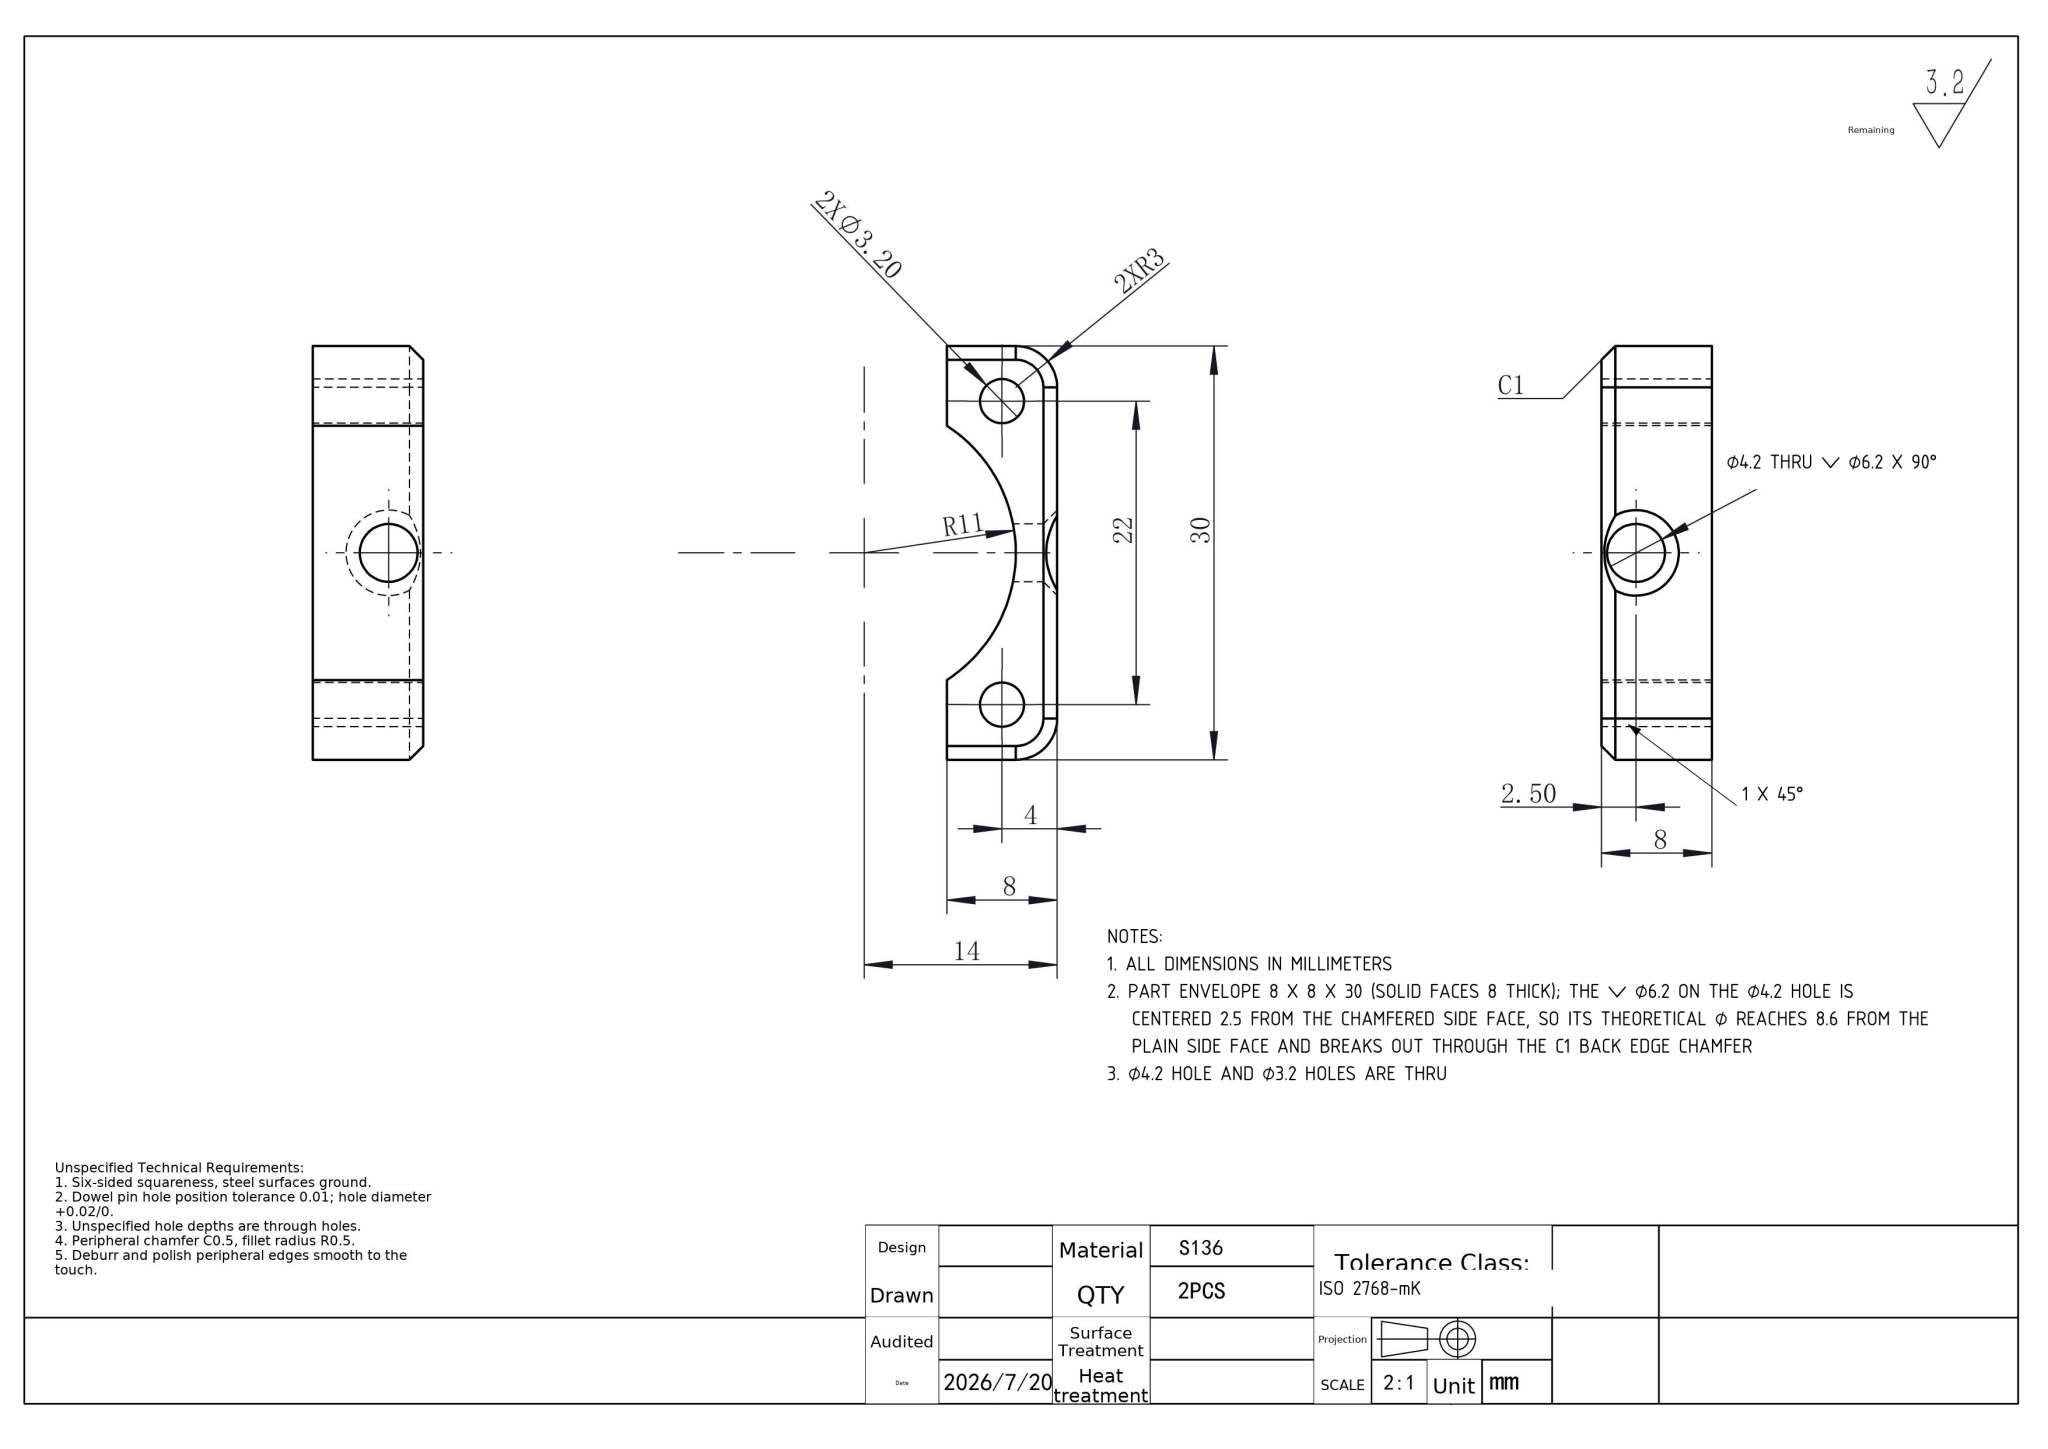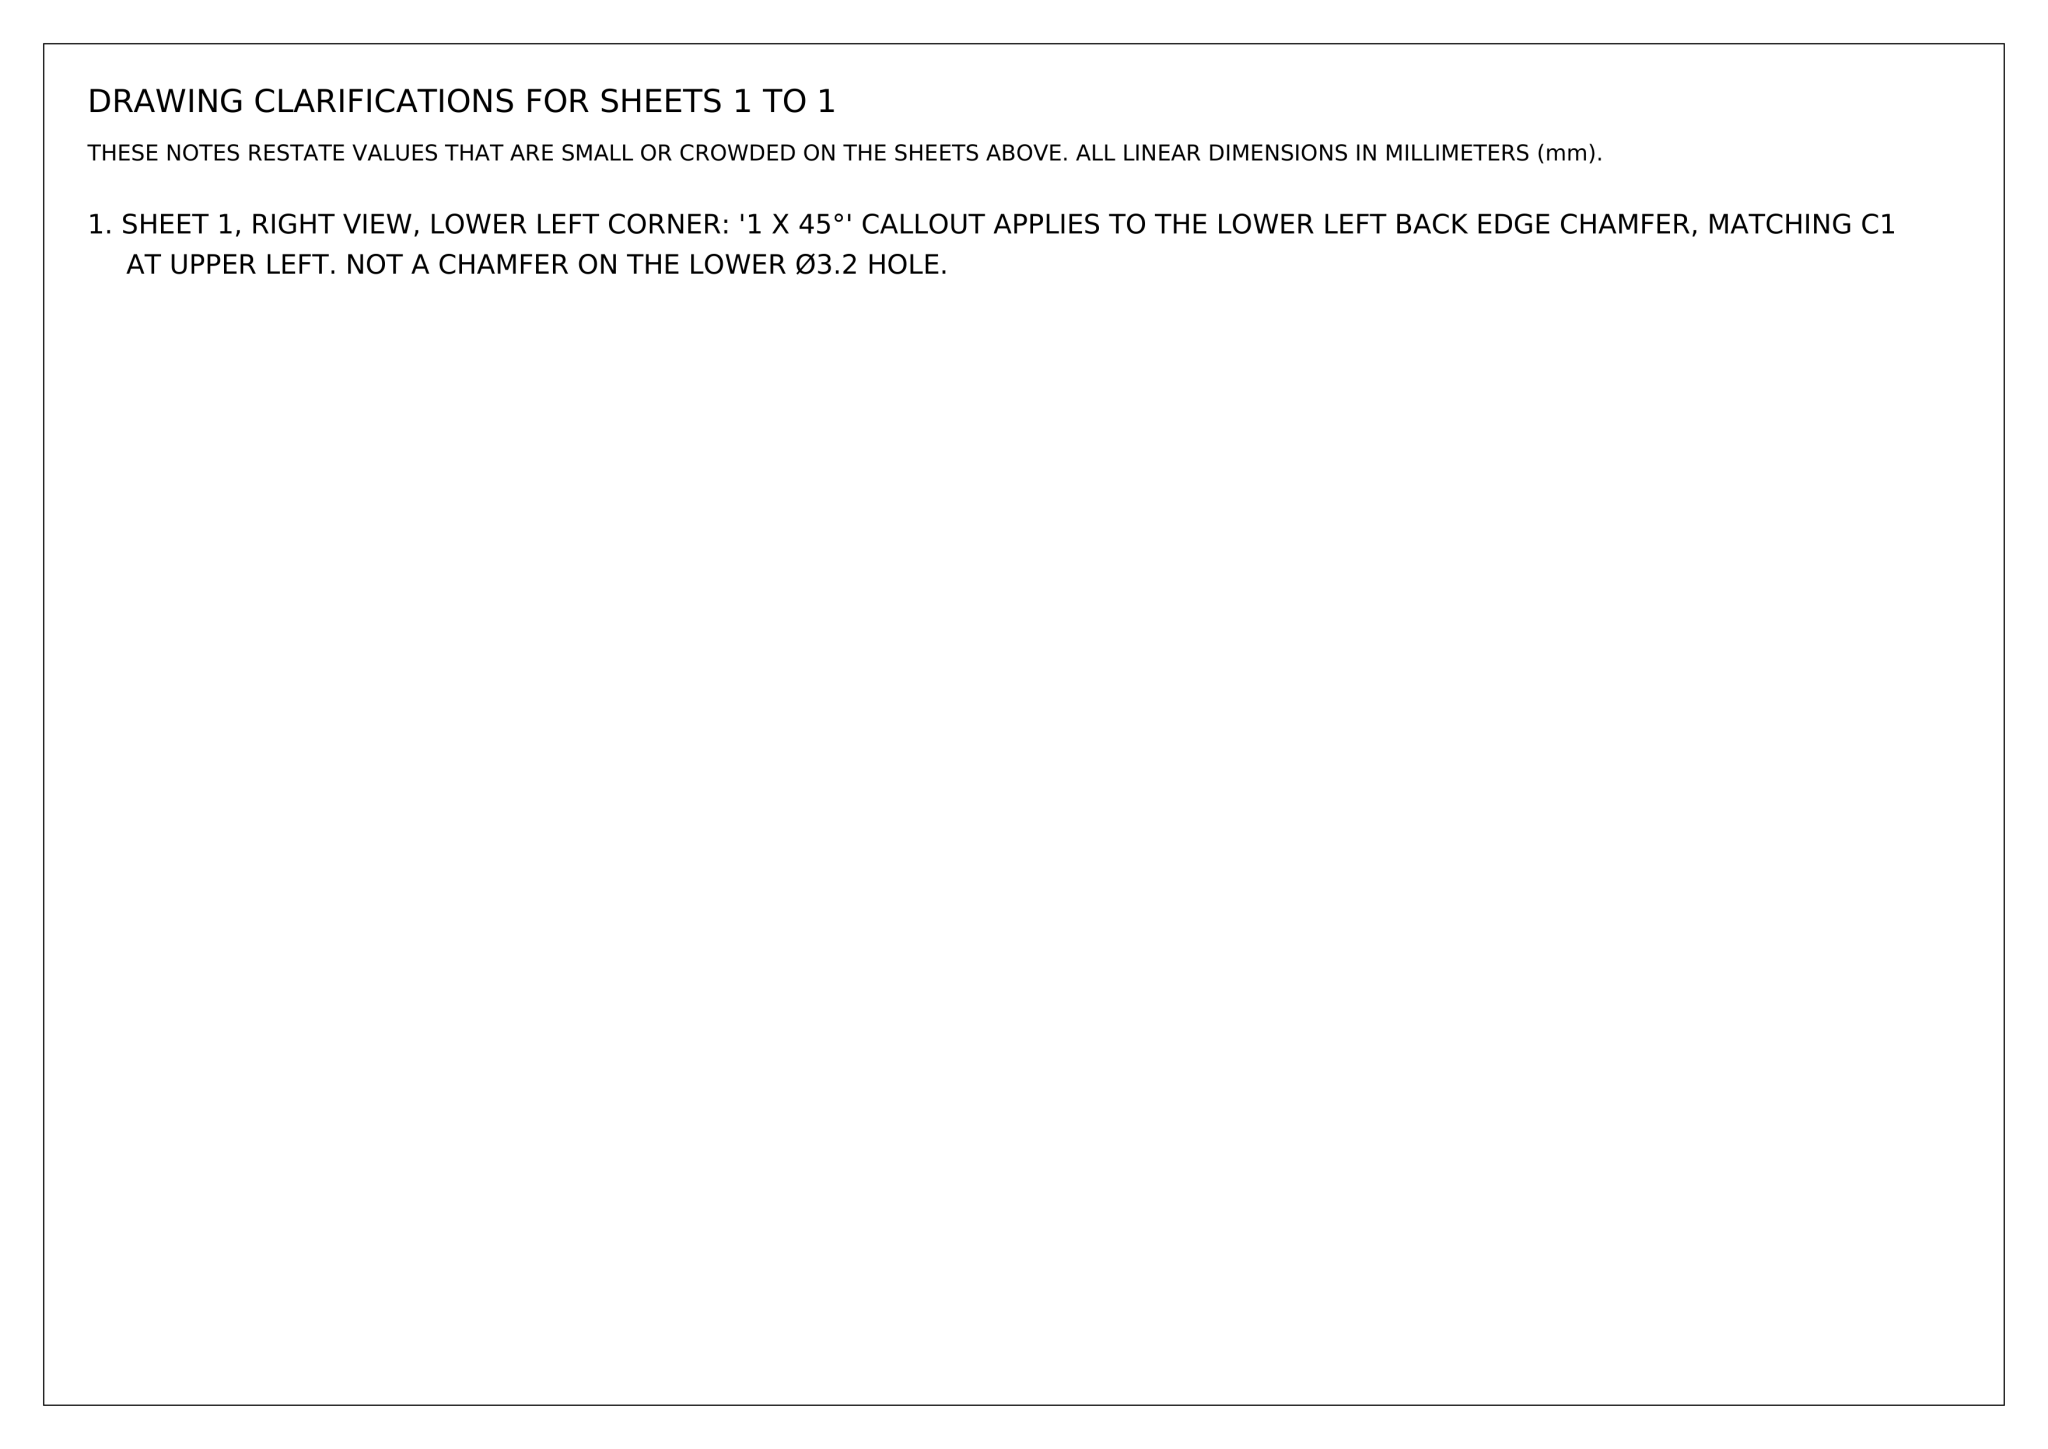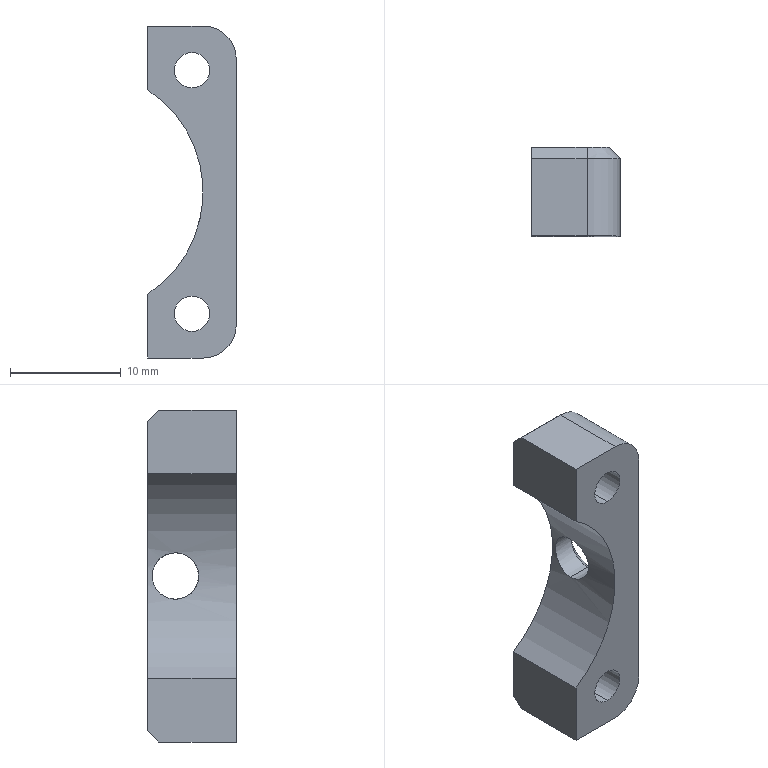Part | NX | mm | 1 solid | 23 faces | box 8 x 8 x 30 mm | volume 1172 mm3 | plane 10 | cylinder 9 | cone 4 | commonest cylinder face diameters 3.2 x4 4.2 x2 6 x2 22 x1
STEP:
#1=COLOUR_RGB('',0.7922,0.8196,0.9333);
#2=FILL_AREA_STYLE_COLOUR('',#1);
#3=FILL_AREA_STYLE('',(#2));
#4=SURFACE_STYLE_FILL_AREA(#3);
#5=SURFACE_SIDE_STYLE('',(#4));
#6=SURFACE_STYLE_USAGE(.BOTH.,#5);
#7=PRESENTATION_STYLE_ASSIGNMENT((#6));
#8=CARTESIAN_POINT('',(13.,5.5,2.1));
#9=VERTEX_POINT('',#8);
#10=CARTESIAN_POINT('',(13.,5.5,-2.1));
#11=VERTEX_POINT('',#10);
#12=CARTESIAN_POINT('',(13.,5.5,0.));
#13=DIRECTION('',(1.,0.,0.));
#14=DIRECTION('',(0.,0.,1.));
#15=AXIS2_PLACEMENT_3D('',#12,#13,#14);
#16=CIRCLE('',#15,2.1);
#17=EDGE_CURVE('',#9,#11,#16,.T.);
#18=ORIENTED_EDGE('',*,*,#17,.F.);
#19=CARTESIAN_POINT('',(14.,5.5,3.1));
#20=VERTEX_POINT('',#19);
#21=CARTESIAN_POINT('',(13.,5.5,2.1));
#22=DIRECTION('',(0.7071,0.,0.7071));
#23=VECTOR('',#22,1000.);
#24=LINE('',#21,#23);
#25=EDGE_CURVE('',#9,#20,#24,.T.);
#26=ORIENTED_EDGE('',*,*,#25,.T.);
#27=CARTESIAN_POINT('',(14.,5.5,-3.1));
#28=VERTEX_POINT('',#27);
#29=CARTESIAN_POINT('',(14.,5.5,0.));
#30=DIRECTION('',(-1.,0.,0.));
#31=DIRECTION('',(0.,0.,1.));
#32=AXIS2_PLACEMENT_3D('',#29,#30,#31);
#33=CIRCLE('',#32,3.1);
#34=EDGE_CURVE('',#28,#20,#33,.T.);
#35=ORIENTED_EDGE('',*,*,#34,.F.);
#36=CARTESIAN_POINT('',(13.,5.5,-2.1));
#37=DIRECTION('',(0.7071,0.,-0.7071));
#38=VECTOR('',#37,1000.);
#39=LINE('',#36,#38);
#40=EDGE_CURVE('',#11,#28,#39,.T.);
#41=ORIENTED_EDGE('',*,*,#40,.F.);
#42=EDGE_LOOP('',(#18,#26,#35,#41));
#43=FACE_OUTER_BOUND('',#42,.T.);
#44=CARTESIAN_POINT('',(13.,5.5,0.));
#45=DIRECTION('',(1.,0.,0.));
#46=DIRECTION('',(0.,0.,-1.));
#47=AXIS2_PLACEMENT_3D('',#44,#45,#46);
#48=CONICAL_SURFACE('',#47,2.1,0.7854);
#49=ADVANCED_FACE('',(#43),#48,.F.);
#50=CARTESIAN_POINT('',(10.798,5.5,2.1));
#51=VERTEX_POINT('',#50);
#52=CARTESIAN_POINT('',(10.798,5.5,-2.1));
#53=VERTEX_POINT('',#52);
#54=CARTESIAN_POINT('',(10.798,5.5,2.1));
#55=CARTESIAN_POINT('',(10.798,5.226,2.1));
#56=CARTESIAN_POINT('',(10.809,4.949,2.045));
#57=CARTESIAN_POINT('',(10.837,4.57,1.888));
#58=CARTESIAN_POINT('',(10.848,4.447,1.822));
#59=CARTESIAN_POINT('',(10.873,4.218,1.669));
#60=CARTESIAN_POINT('',(10.886,4.113,1.583));
#61=CARTESIAN_POINT('',(10.912,3.919,1.389));
#62=CARTESIAN_POINT('',(10.926,3.831,1.281));
#63=CARTESIAN_POINT('',(10.95,3.678,1.054));
#64=CARTESIAN_POINT('',(10.961,3.614,0.9335));
#65=CARTESIAN_POINT('',(10.989,3.455,0.5515));
#66=CARTESIAN_POINT('',(11.,3.4,0.2784));
#67=CARTESIAN_POINT('',(11.,3.4,-0.1376));
#68=CARTESIAN_POINT('',(10.997,3.413,-0.2741));
#69=CARTESIAN_POINT('',(10.987,3.467,-0.5432));
#70=CARTESIAN_POINT('',(10.98,3.507,-0.677));
#71=CARTESIAN_POINT('',(10.961,3.613,-0.9308));
#72=CARTESIAN_POINT('',(10.95,3.677,-1.051));
#73=CARTESIAN_POINT('',(10.926,3.829,-1.28));
#74=CARTESIAN_POINT('',(10.913,3.918,-1.387));
#75=CARTESIAN_POINT('',(10.873,4.207,-1.677));
#76=CARTESIAN_POINT('',(10.847,4.441,-1.834));
#77=CARTESIAN_POINT('',(10.818,4.819,-1.991));
#78=CARTESIAN_POINT('',(10.811,4.953,-2.032));
#79=CARTESIAN_POINT('',(10.8,5.224,-2.086));
#80=CARTESIAN_POINT('',(10.798,5.361,-2.1));
#81=CARTESIAN_POINT('',(10.798,5.5,-2.1));
#82=B_SPLINE_CURVE_WITH_KNOTS('',3,(#54,#55,#56,#57,#58,#59,#60,#61,#62,#63,#64,#65,#66,#67,#68,#69,#70,#71,#72,#73,#74,#75,#76,#77,#78,#79,#80,#81),.UNSPECIFIED.,.F.,.F.,(4,2,2,2,2,2,2,2,2,2,2,2,2,4),(0.006581,0.007403,0.007814,0.008225,0.008637,0.009048,0.00987,0.01028,0.01069,0.0111,0.01151,0.01234,0.01275,0.01316),.UNSPECIFIED.);
#83=EDGE_CURVE('',#51,#53,#82,.T.);
#84=ORIENTED_EDGE('',*,*,#83,.F.);
#85=CARTESIAN_POINT('',(6.,5.5,2.1));
#86=DIRECTION('',(1.,0.,0.));
#87=VECTOR('',#86,1000.);
#88=LINE('',#85,#87);
#89=EDGE_CURVE('',#51,#9,#88,.T.);
#90=ORIENTED_EDGE('',*,*,#89,.T.);
#91=ORIENTED_EDGE('',*,*,#17,.T.);
#92=CARTESIAN_POINT('',(6.,5.5,-2.1));
#93=DIRECTION('',(1.,0.,0.));
#94=VECTOR('',#93,1000.);
#95=LINE('',#92,#94);
#96=EDGE_CURVE('',#53,#11,#95,.T.);
#97=ORIENTED_EDGE('',*,*,#96,.F.);
#98=EDGE_LOOP('',(#84,#90,#91,#97));
#99=FACE_OUTER_BOUND('',#98,.T.);
#100=CARTESIAN_POINT('',(6.,5.5,0.));
#101=DIRECTION('',(1.,0.,0.));
#102=DIRECTION('',(0.,0.,-1.));
#103=AXIS2_PLACEMENT_3D('',#100,#101,#102);
#104=CYLINDRICAL_SURFACE('',#103,2.1);
#105=ADVANCED_FACE('',(#99),#104,.F.);
#106=CARTESIAN_POINT('',(10.,0.,-12.6));
#107=VERTEX_POINT('',#106);
#108=CARTESIAN_POINT('',(10.,0.,-9.4));
#109=VERTEX_POINT('',#108);
#110=CARTESIAN_POINT('',(10.,0.,-11.));
#111=DIRECTION('',(0.,1.,0.));
#112=DIRECTION('',(0.,0.,1.));
#113=AXIS2_PLACEMENT_3D('',#110,#111,#112);
#114=CIRCLE('',#113,1.6);
#115=EDGE_CURVE('',#107,#109,#114,.T.);
#116=ORIENTED_EDGE('',*,*,#115,.F.);
#117=CARTESIAN_POINT('',(10.,8.,-12.6));
#118=VERTEX_POINT('',#117);
#119=CARTESIAN_POINT('',(10.,0.,-12.6));
#120=DIRECTION('',(0.,1.,0.));
#121=VECTOR('',#120,1000.);
#122=LINE('',#119,#121);
#123=EDGE_CURVE('',#107,#118,#122,.T.);
#124=ORIENTED_EDGE('',*,*,#123,.T.);
#125=CARTESIAN_POINT('',(10.,8.,-9.4));
#126=VERTEX_POINT('',#125);
#127=CARTESIAN_POINT('',(10.,8.,-11.));
#128=DIRECTION('',(0.,1.,0.));
#129=DIRECTION('',(0.,0.,1.));
#130=AXIS2_PLACEMENT_3D('',#127,#128,#129);
#131=CIRCLE('',#130,1.6);
#132=EDGE_CURVE('',#118,#126,#131,.T.);
#133=ORIENTED_EDGE('',*,*,#132,.T.);
#134=CARTESIAN_POINT('',(10.,0.,-9.4));
#135=DIRECTION('',(0.,1.,0.));
#136=VECTOR('',#135,1000.);
#137=LINE('',#134,#136);
#138=EDGE_CURVE('',#109,#126,#137,.T.);
#139=ORIENTED_EDGE('',*,*,#138,.F.);
#140=EDGE_LOOP('',(#116,#124,#133,#139));
#141=FACE_OUTER_BOUND('',#140,.T.);
#142=CARTESIAN_POINT('',(10.,0.,-11.));
#143=DIRECTION('',(0.,1.,0.));
#144=DIRECTION('',(0.,0.,1.));
#145=AXIS2_PLACEMENT_3D('',#142,#143,#144);
#146=CYLINDRICAL_SURFACE('',#145,1.6);
#147=ADVANCED_FACE('',(#141),#146,.F.);
#148=CARTESIAN_POINT('',(10.,0.,9.4));
#149=VERTEX_POINT('',#148);
#150=CARTESIAN_POINT('',(10.,0.,12.6));
#151=VERTEX_POINT('',#150);
#152=CARTESIAN_POINT('',(10.,0.,11.));
#153=DIRECTION('',(0.,1.,0.));
#154=DIRECTION('',(0.,0.,1.));
#155=AXIS2_PLACEMENT_3D('',#152,#153,#154);
#156=CIRCLE('',#155,1.6);
#157=EDGE_CURVE('',#149,#151,#156,.T.);
#158=ORIENTED_EDGE('',*,*,#157,.F.);
#159=CARTESIAN_POINT('',(10.,8.,9.4));
#160=VERTEX_POINT('',#159);
#161=CARTESIAN_POINT('',(10.,0.,9.4));
#162=DIRECTION('',(0.,1.,0.));
#163=VECTOR('',#162,1000.);
#164=LINE('',#161,#163);
#165=EDGE_CURVE('',#149,#160,#164,.T.);
#166=ORIENTED_EDGE('',*,*,#165,.T.);
#167=CARTESIAN_POINT('',(10.,8.,12.6));
#168=VERTEX_POINT('',#167);
#169=CARTESIAN_POINT('',(10.,8.,11.));
#170=DIRECTION('',(0.,1.,0.));
#171=DIRECTION('',(0.,0.,1.));
#172=AXIS2_PLACEMENT_3D('',#169,#170,#171);
#173=CIRCLE('',#172,1.6);
#174=EDGE_CURVE('',#160,#168,#173,.T.);
#175=ORIENTED_EDGE('',*,*,#174,.T.);
#176=CARTESIAN_POINT('',(10.,0.,12.6));
#177=DIRECTION('',(0.,1.,0.));
#178=VECTOR('',#177,1000.);
#179=LINE('',#176,#178);
#180=EDGE_CURVE('',#151,#168,#179,.T.);
#181=ORIENTED_EDGE('',*,*,#180,.F.);
#182=EDGE_LOOP('',(#158,#166,#175,#181));
#183=FACE_OUTER_BOUND('',#182,.T.);
#184=CARTESIAN_POINT('',(10.,0.,11.));
#185=DIRECTION('',(0.,1.,0.));
#186=DIRECTION('',(0.,0.,1.));
#187=AXIS2_PLACEMENT_3D('',#184,#185,#186);
#188=CYLINDRICAL_SURFACE('',#187,1.6);
#189=ADVANCED_FACE('',(#183),#188,.F.);
#190=CARTESIAN_POINT('',(14.,7.,-12.));
#191=VERTEX_POINT('',#190);
#192=CARTESIAN_POINT('',(14.,7.,-2.713));
#193=VERTEX_POINT('',#192);
#194=CARTESIAN_POINT('',(14.,7.,12.));
#195=DIRECTION('',(0.,0.,1.));
#196=VECTOR('',#195,1000.);
#197=LINE('',#194,#196);
#198=EDGE_CURVE('',#191,#193,#197,.T.);
#199=ORIENTED_EDGE('',*,*,#198,.T.);
#200=CARTESIAN_POINT('',(14.,5.5,0.));
#201=DIRECTION('',(-1.,0.,0.));
#202=DIRECTION('',(0.,0.,1.));
#203=AXIS2_PLACEMENT_3D('',#200,#201,#202);
#204=CIRCLE('',#203,3.1);
#205=EDGE_CURVE('',#193,#28,#204,.T.);
#206=ORIENTED_EDGE('',*,*,#205,.T.);
#207=ORIENTED_EDGE('',*,*,#34,.T.);
#208=CARTESIAN_POINT('',(14.,7.,2.713));
#209=VERTEX_POINT('',#208);
#210=CARTESIAN_POINT('',(14.,5.5,0.));
#211=DIRECTION('',(-1.,0.,0.));
#212=DIRECTION('',(0.,0.,1.));
#213=AXIS2_PLACEMENT_3D('',#210,#211,#212);
#214=CIRCLE('',#213,3.1);
#215=EDGE_CURVE('',#20,#209,#214,.T.);
#216=ORIENTED_EDGE('',*,*,#215,.T.);
#217=CARTESIAN_POINT('',(14.,7.,12.));
#218=VERTEX_POINT('',#217);
#219=CARTESIAN_POINT('',(14.,7.,12.));
#220=DIRECTION('',(0.,0.,1.));
#221=VECTOR('',#220,1000.);
#222=LINE('',#219,#221);
#223=EDGE_CURVE('',#209,#218,#222,.T.);
#224=ORIENTED_EDGE('',*,*,#223,.T.);
#225=CARTESIAN_POINT('',(14.,0.,12.));
#226=VERTEX_POINT('',#225);
#227=CARTESIAN_POINT('',(14.,8.,12.));
#228=DIRECTION('',(0.,-1.,0.));
#229=VECTOR('',#228,1000.);
#230=LINE('',#227,#229);
#231=EDGE_CURVE('',#218,#226,#230,.T.);
#232=ORIENTED_EDGE('',*,*,#231,.T.);
#233=CARTESIAN_POINT('',(14.,0.,-12.));
#234=VERTEX_POINT('',#233);
#235=CARTESIAN_POINT('',(14.,0.,-15.));
#236=DIRECTION('',(0.,0.,-1.));
#237=VECTOR('',#236,1000.);
#238=LINE('',#235,#237);
#239=EDGE_CURVE('',#226,#234,#238,.T.);
#240=ORIENTED_EDGE('',*,*,#239,.T.);
#241=CARTESIAN_POINT('',(14.,8.,-12.));
#242=DIRECTION('',(0.,1.,0.));
#243=VECTOR('',#242,1000.);
#244=LINE('',#241,#243);
#245=EDGE_CURVE('',#234,#191,#244,.T.);
#246=ORIENTED_EDGE('',*,*,#245,.T.);
#247=EDGE_LOOP('',(#199,#206,#207,#216,#224,#232,#240,#246));
#248=FACE_OUTER_BOUND('',#247,.T.);
#249=CARTESIAN_POINT('',(14.,8.,-15.));
#250=DIRECTION('',(-1.,0.,0.));
#251=DIRECTION('',(0.,0.,1.));
#252=AXIS2_PLACEMENT_3D('',#249,#250,#251);
#253=PLANE('',#252);
#254=ADVANCED_FACE('',(#248),#253,.F.);
#255=CARTESIAN_POINT('',(6.,7.,-15.));
#256=VERTEX_POINT('',#255);
#257=CARTESIAN_POINT('',(6.,0.,-15.));
#258=VERTEX_POINT('',#257);
#259=CARTESIAN_POINT('',(6.,8.,-15.));
#260=DIRECTION('',(0.,-1.,0.));
#261=VECTOR('',#260,1000.);
#262=LINE('',#259,#261);
#263=EDGE_CURVE('',#256,#258,#262,.T.);
#264=ORIENTED_EDGE('',*,*,#263,.F.);
#265=CARTESIAN_POINT('',(11.,7.,-15.));
#266=VERTEX_POINT('',#265);
#267=CARTESIAN_POINT('',(11.,7.,-15.));
#268=DIRECTION('',(1.,0.,0.));
#269=VECTOR('',#268,1000.);
#270=LINE('',#267,#269);
#271=EDGE_CURVE('',#256,#266,#270,.T.);
#272=ORIENTED_EDGE('',*,*,#271,.T.);
#273=CARTESIAN_POINT('',(11.,0.,-15.));
#274=VERTEX_POINT('',#273);
#275=CARTESIAN_POINT('',(11.,8.,-15.));
#276=DIRECTION('',(0.,-1.,0.));
#277=VECTOR('',#276,1000.);
#278=LINE('',#275,#277);
#279=EDGE_CURVE('',#266,#274,#278,.T.);
#280=ORIENTED_EDGE('',*,*,#279,.T.);
#281=CARTESIAN_POINT('',(6.,0.,-15.));
#282=DIRECTION('',(-1.,0.,0.));
#283=VECTOR('',#282,1000.);
#284=LINE('',#281,#283);
#285=EDGE_CURVE('',#274,#258,#284,.T.);
#286=ORIENTED_EDGE('',*,*,#285,.T.);
#287=EDGE_LOOP('',(#264,#272,#280,#286));
#288=FACE_OUTER_BOUND('',#287,.T.);
#289=CARTESIAN_POINT('',(6.,8.,-15.));
#290=DIRECTION('',(0.,0.,1.));
#291=DIRECTION('',(1.,0.,0.));
#292=AXIS2_PLACEMENT_3D('',#289,#290,#291);
#293=PLANE('',#292);
#294=ADVANCED_FACE('',(#288),#293,.F.);
#295=CARTESIAN_POINT('',(6.,8.,-14.));
#296=VERTEX_POINT('',#295);
#297=CARTESIAN_POINT('',(6.,8.,-9.22));
#298=VERTEX_POINT('',#297);
#299=CARTESIAN_POINT('',(6.,8.,-15.));
#300=DIRECTION('',(0.,0.,1.));
#301=VECTOR('',#300,1000.);
#302=LINE('',#299,#301);
#303=EDGE_CURVE('',#296,#298,#302,.T.);
#304=ORIENTED_EDGE('',*,*,#303,.F.);
#305=CARTESIAN_POINT('',(6.,8.,-14.));
#306=DIRECTION('',(0.,-0.7071,-0.7071));
#307=VECTOR('',#306,1000.);
#308=LINE('',#305,#307);
#309=EDGE_CURVE('',#296,#256,#308,.T.);
#310=ORIENTED_EDGE('',*,*,#309,.T.);
#311=ORIENTED_EDGE('',*,*,#263,.T.);
#312=CARTESIAN_POINT('',(6.,0.,-9.22));
#313=VERTEX_POINT('',#312);
#314=CARTESIAN_POINT('',(6.,0.,-15.));
#315=DIRECTION('',(0.,0.,1.));
#316=VECTOR('',#315,1000.);
#317=LINE('',#314,#316);
#318=EDGE_CURVE('',#258,#313,#317,.T.);
#319=ORIENTED_EDGE('',*,*,#318,.T.);
#320=CARTESIAN_POINT('',(6.,8.,-9.22));
#321=DIRECTION('',(0.,-1.,0.));
#322=VECTOR('',#321,1000.);
#323=LINE('',#320,#322);
#324=EDGE_CURVE('',#298,#313,#323,.T.);
#325=ORIENTED_EDGE('',*,*,#324,.F.);
#326=EDGE_LOOP('',(#304,#310,#311,#319,#325));
#327=FACE_OUTER_BOUND('',#326,.T.);
#328=CARTESIAN_POINT('',(6.,8.,-15.));
#329=DIRECTION('',(1.,0.,0.));
#330=DIRECTION('',(0.,0.,-1.));
#331=AXIS2_PLACEMENT_3D('',#328,#329,#330);
#332=PLANE('',#331);
#333=ADVANCED_FACE('',(#327),#332,.F.);
#334=CARTESIAN_POINT('',(10.798,5.5,-2.1));
#335=CARTESIAN_POINT('',(10.798,5.639,-2.1));
#336=CARTESIAN_POINT('',(10.8,5.776,-2.086));
#337=CARTESIAN_POINT('',(10.811,6.045,-2.033));
#338=CARTESIAN_POINT('',(10.818,6.178,-1.992));
#339=CARTESIAN_POINT('',(10.837,6.432,-1.887));
#340=CARTESIAN_POINT('',(10.848,6.553,-1.822));
#341=CARTESIAN_POINT('',(10.873,6.781,-1.67));
#342=CARTESIAN_POINT('',(10.886,6.889,-1.581));
#343=CARTESIAN_POINT('',(10.926,7.178,-1.291));
#344=CARTESIAN_POINT('',(10.952,7.335,-1.057));
#345=CARTESIAN_POINT('',(10.989,7.544,-0.5523));
#346=CARTESIAN_POINT('',(11.,7.6,-0.2755));
#347=CARTESIAN_POINT('',(11.,7.6,0.1365));
#348=CARTESIAN_POINT('',(10.997,7.586,0.276));
#349=CARTESIAN_POINT('',(10.987,7.533,0.5456));
#350=CARTESIAN_POINT('',(10.98,7.493,0.6767));
#351=CARTESIAN_POINT('',(10.961,7.387,0.9314));
#352=CARTESIAN_POINT('',(10.95,7.322,1.054));
#353=CARTESIAN_POINT('',(10.926,7.17,1.281));
#354=CARTESIAN_POINT('',(10.913,7.082,1.387));
#355=CARTESIAN_POINT('',(10.886,6.887,1.583));
#356=CARTESIAN_POINT('',(10.873,6.781,1.669));
#357=CARTESIAN_POINT('',(10.848,6.554,1.821));
#358=CARTESIAN_POINT('',(10.837,6.431,1.887));
#359=CARTESIAN_POINT('',(10.818,6.177,1.992));
#360=CARTESIAN_POINT('',(10.811,6.046,2.032));
#361=CARTESIAN_POINT('',(10.8,5.777,2.086));
#362=CARTESIAN_POINT('',(10.798,5.637,2.1));
#363=CARTESIAN_POINT('',(10.798,5.5,2.1));
#364=B_SPLINE_CURVE_WITH_KNOTS('',3,(#334,#335,#336,#337,#338,#339,#340,#341,#342,#343,#344,#345,#346,#347,#348,#349,#350,#351,#352,#353,#354,#355,#356,#357,#358,#359,#360,#361,#362,#363),.UNSPECIFIED.,.F.,.F.,(4,2,2,2,2,2,2,2,2,2,2,2,2,2,4),(0.,0.0004113,0.0008226,0.001234,0.001645,0.002468,0.00329,0.003702,0.004113,0.004524,0.004935,0.005347,0.005758,0.006169,0.006581),.UNSPECIFIED.);
#365=EDGE_CURVE('',#53,#51,#364,.T.);
#366=ORIENTED_EDGE('',*,*,#365,.T.);
#367=ORIENTED_EDGE('',*,*,#83,.T.);
#368=EDGE_LOOP('',(#366,#367));
#369=FACE_BOUND('',#368,.T.);
#370=CARTESIAN_POINT('',(6.,0.,9.22));
#371=VERTEX_POINT('',#370);
#372=CARTESIAN_POINT('',(0.,0.,0.));
#373=DIRECTION('',(0.,-1.,0.));
#374=DIRECTION('',(0.,0.,1.));
#375=AXIS2_PLACEMENT_3D('',#372,#373,#374);
#376=CIRCLE('',#375,11.);
#377=EDGE_CURVE('',#313,#371,#376,.T.);
#378=ORIENTED_EDGE('',*,*,#377,.T.);
#379=CARTESIAN_POINT('',(6.,8.,9.22));
#380=VERTEX_POINT('',#379);
#381=CARTESIAN_POINT('',(6.,8.,9.22));
#382=DIRECTION('',(0.,-1.,0.));
#383=VECTOR('',#382,1000.);
#384=LINE('',#381,#383);
#385=EDGE_CURVE('',#380,#371,#384,.T.);
#386=ORIENTED_EDGE('',*,*,#385,.F.);
#387=CARTESIAN_POINT('',(0.,8.,0.));
#388=DIRECTION('',(0.,-1.,0.));
#389=DIRECTION('',(0.,0.,1.));
#390=AXIS2_PLACEMENT_3D('',#387,#388,#389);
#391=CIRCLE('',#390,11.);
#392=EDGE_CURVE('',#298,#380,#391,.T.);
#393=ORIENTED_EDGE('',*,*,#392,.F.);
#394=ORIENTED_EDGE('',*,*,#324,.T.);
#395=EDGE_LOOP('',(#378,#386,#393,#394));
#396=FACE_OUTER_BOUND('',#395,.T.);
#397=CARTESIAN_POINT('',(0.,8.,0.));
#398=DIRECTION('',(0.,-1.,0.));
#399=DIRECTION('',(0.,0.,-1.));
#400=AXIS2_PLACEMENT_3D('',#397,#398,#399);
#401=CYLINDRICAL_SURFACE('',#400,11.);
#402=ADVANCED_FACE('',(#369,#396),#401,.F.);
#403=CARTESIAN_POINT('',(6.,7.,15.));
#404=VERTEX_POINT('',#403);
#405=CARTESIAN_POINT('',(6.,0.,15.));
#406=VERTEX_POINT('',#405);
#407=CARTESIAN_POINT('',(6.,8.,15.));
#408=DIRECTION('',(0.,-1.,0.));
#409=VECTOR('',#408,1000.);
#410=LINE('',#407,#409);
#411=EDGE_CURVE('',#404,#406,#410,.T.);
#412=ORIENTED_EDGE('',*,*,#411,.F.);
#413=CARTESIAN_POINT('',(6.,8.,14.));
#414=VERTEX_POINT('',#413);
#415=CARTESIAN_POINT('',(6.,8.,14.));
#416=DIRECTION('',(0.,0.7071,-0.7071));
#417=VECTOR('',#416,1000.);
#418=LINE('',#415,#417);
#419=EDGE_CURVE('',#404,#414,#418,.T.);
#420=ORIENTED_EDGE('',*,*,#419,.T.);
#421=CARTESIAN_POINT('',(6.,8.,9.22));
#422=DIRECTION('',(0.,0.,1.));
#423=VECTOR('',#422,1000.);
#424=LINE('',#421,#423);
#425=EDGE_CURVE('',#380,#414,#424,.T.);
#426=ORIENTED_EDGE('',*,*,#425,.F.);
#427=ORIENTED_EDGE('',*,*,#385,.T.);
#428=CARTESIAN_POINT('',(6.,0.,9.22));
#429=DIRECTION('',(0.,0.,1.));
#430=VECTOR('',#429,1000.);
#431=LINE('',#428,#430);
#432=EDGE_CURVE('',#371,#406,#431,.T.);
#433=ORIENTED_EDGE('',*,*,#432,.T.);
#434=EDGE_LOOP('',(#412,#420,#426,#427,#433));
#435=FACE_OUTER_BOUND('',#434,.T.);
#436=CARTESIAN_POINT('',(6.,8.,9.22));
#437=DIRECTION('',(1.,0.,0.));
#438=DIRECTION('',(0.,0.,-1.));
#439=AXIS2_PLACEMENT_3D('',#436,#437,#438);
#440=PLANE('',#439);
#441=ADVANCED_FACE('',(#435),#440,.F.);
#442=CARTESIAN_POINT('',(11.,0.,15.));
#443=VERTEX_POINT('',#442);
#444=CARTESIAN_POINT('',(11.,7.,15.));
#445=VERTEX_POINT('',#444);
#446=CARTESIAN_POINT('',(11.,8.,15.));
#447=DIRECTION('',(0.,1.,0.));
#448=VECTOR('',#447,1000.);
#449=LINE('',#446,#448);
#450=EDGE_CURVE('',#443,#445,#449,.T.);
#451=ORIENTED_EDGE('',*,*,#450,.T.);
#452=CARTESIAN_POINT('',(6.,7.,15.));
#453=DIRECTION('',(-1.,0.,0.));
#454=VECTOR('',#453,1000.);
#455=LINE('',#452,#454);
#456=EDGE_CURVE('',#445,#404,#455,.T.);
#457=ORIENTED_EDGE('',*,*,#456,.T.);
#458=ORIENTED_EDGE('',*,*,#411,.T.);
#459=CARTESIAN_POINT('',(14.,0.,15.));
#460=DIRECTION('',(1.,0.,0.));
#461=VECTOR('',#460,1000.);
#462=LINE('',#459,#461);
#463=EDGE_CURVE('',#406,#443,#462,.T.);
#464=ORIENTED_EDGE('',*,*,#463,.T.);
#465=EDGE_LOOP('',(#451,#457,#458,#464));
#466=FACE_OUTER_BOUND('',#465,.T.);
#467=CARTESIAN_POINT('',(14.,8.,15.));
#468=DIRECTION('',(0.,0.,-1.));
#469=DIRECTION('',(-1.,0.,0.));
#470=AXIS2_PLACEMENT_3D('',#467,#468,#469);
#471=PLANE('',#470);
#472=ADVANCED_FACE('',(#466),#471,.F.);
#473=CARTESIAN_POINT('',(10.,8.,-11.));
#474=DIRECTION('',(0.,1.,0.));
#475=DIRECTION('',(0.,0.,1.));
#476=AXIS2_PLACEMENT_3D('',#473,#474,#475);
#477=CIRCLE('',#476,1.6);
#478=EDGE_CURVE('',#126,#118,#477,.T.);
#479=ORIENTED_EDGE('',*,*,#478,.F.);
#480=ORIENTED_EDGE('',*,*,#132,.F.);
#481=EDGE_LOOP('',(#479,#480));
#482=FACE_BOUND('',#481,.T.);
#483=CARTESIAN_POINT('',(10.,8.,11.));
#484=DIRECTION('',(0.,1.,0.));
#485=DIRECTION('',(0.,0.,1.));
#486=AXIS2_PLACEMENT_3D('',#483,#484,#485);
#487=CIRCLE('',#486,1.6);
#488=EDGE_CURVE('',#168,#160,#487,.T.);
#489=ORIENTED_EDGE('',*,*,#488,.F.);
#490=ORIENTED_EDGE('',*,*,#174,.F.);
#491=EDGE_LOOP('',(#489,#490));
#492=FACE_BOUND('',#491,.T.);
#493=ORIENTED_EDGE('',*,*,#425,.T.);
#494=CARTESIAN_POINT('',(11.,8.,14.));
#495=VERTEX_POINT('',#494);
#496=CARTESIAN_POINT('',(11.,8.,14.));
#497=DIRECTION('',(1.,0.,0.));
#498=VECTOR('',#497,1000.);
#499=LINE('',#496,#498);
#500=EDGE_CURVE('',#414,#495,#499,.T.);
#501=ORIENTED_EDGE('',*,*,#500,.T.);
#502=CARTESIAN_POINT('',(13.,8.,12.));
#503=VERTEX_POINT('',#502);
#504=CARTESIAN_POINT('',(11.,8.,12.));
#505=DIRECTION('',(0.,1.,0.));
#506=DIRECTION('',(0.,0.,1.));
#507=AXIS2_PLACEMENT_3D('',#504,#505,#506);
#508=CIRCLE('',#507,2.);
#509=EDGE_CURVE('',#495,#503,#508,.T.);
#510=ORIENTED_EDGE('',*,*,#509,.T.);
#511=CARTESIAN_POINT('',(13.,8.,-12.));
#512=VERTEX_POINT('',#511);
#513=CARTESIAN_POINT('',(13.,8.,-12.));
#514=DIRECTION('',(0.,0.,-1.));
#515=VECTOR('',#514,1000.);
#516=LINE('',#513,#515);
#517=EDGE_CURVE('',#503,#512,#516,.T.);
#518=ORIENTED_EDGE('',*,*,#517,.T.);
#519=CARTESIAN_POINT('',(11.,8.,-14.));
#520=VERTEX_POINT('',#519);
#521=CARTESIAN_POINT('',(11.,8.,-12.));
#522=DIRECTION('',(0.,1.,0.));
#523=DIRECTION('',(0.,0.,1.));
#524=AXIS2_PLACEMENT_3D('',#521,#522,#523);
#525=CIRCLE('',#524,2.);
#526=EDGE_CURVE('',#512,#520,#525,.T.);
#527=ORIENTED_EDGE('',*,*,#526,.T.);
#528=CARTESIAN_POINT('',(6.,8.,-14.));
#529=DIRECTION('',(-1.,0.,0.));
#530=VECTOR('',#529,1000.);
#531=LINE('',#528,#530);
#532=EDGE_CURVE('',#520,#296,#531,.T.);
#533=ORIENTED_EDGE('',*,*,#532,.T.);
#534=ORIENTED_EDGE('',*,*,#303,.T.);
#535=ORIENTED_EDGE('',*,*,#392,.T.);
#536=EDGE_LOOP('',(#493,#501,#510,#518,#527,#533,#534,#535));
#537=FACE_OUTER_BOUND('',#536,.T.);
#538=CARTESIAN_POINT('',(0.,8.,0.));
#539=DIRECTION('',(0.,1.,0.));
#540=DIRECTION('',(0.,0.,1.));
#541=AXIS2_PLACEMENT_3D('',#538,#539,#540);
#542=PLANE('',#541);
#543=ADVANCED_FACE('',(#482,#492,#537),#542,.T.);
#544=CARTESIAN_POINT('',(10.,0.,-11.));
#545=DIRECTION('',(0.,1.,0.));
#546=DIRECTION('',(0.,0.,1.));
#547=AXIS2_PLACEMENT_3D('',#544,#545,#546);
#548=CIRCLE('',#547,1.6);
#549=EDGE_CURVE('',#109,#107,#548,.T.);
#550=ORIENTED_EDGE('',*,*,#549,.T.);
#551=ORIENTED_EDGE('',*,*,#115,.T.);
#552=EDGE_LOOP('',(#550,#551));
#553=FACE_BOUND('',#552,.T.);
#554=CARTESIAN_POINT('',(10.,0.,11.));
#555=DIRECTION('',(0.,1.,0.));
#556=DIRECTION('',(0.,0.,1.));
#557=AXIS2_PLACEMENT_3D('',#554,#555,#556);
#558=CIRCLE('',#557,1.6);
#559=EDGE_CURVE('',#151,#149,#558,.T.);
#560=ORIENTED_EDGE('',*,*,#559,.T.);
#561=ORIENTED_EDGE('',*,*,#157,.T.);
#562=EDGE_LOOP('',(#560,#561));
#563=FACE_BOUND('',#562,.T.);
#564=ORIENTED_EDGE('',*,*,#285,.F.);
#565=CARTESIAN_POINT('',(11.,0.,-12.));
#566=DIRECTION('',(0.,-1.,0.));
#567=DIRECTION('',(0.,0.,1.));
#568=AXIS2_PLACEMENT_3D('',#565,#566,#567);
#569=CIRCLE('',#568,3.);
#570=EDGE_CURVE('',#274,#234,#569,.T.);
#571=ORIENTED_EDGE('',*,*,#570,.T.);
#572=ORIENTED_EDGE('',*,*,#239,.F.);
#573=CARTESIAN_POINT('',(11.,0.,12.));
#574=DIRECTION('',(0.,-1.,0.));
#575=DIRECTION('',(0.,0.,1.));
#576=AXIS2_PLACEMENT_3D('',#573,#574,#575);
#577=CIRCLE('',#576,3.);
#578=EDGE_CURVE('',#226,#443,#577,.T.);
#579=ORIENTED_EDGE('',*,*,#578,.T.);
#580=ORIENTED_EDGE('',*,*,#463,.F.);
#581=ORIENTED_EDGE('',*,*,#432,.F.);
#582=ORIENTED_EDGE('',*,*,#377,.F.);
#583=ORIENTED_EDGE('',*,*,#318,.F.);
#584=EDGE_LOOP('',(#564,#571,#572,#579,#580,#581,#582,#583));
#585=FACE_OUTER_BOUND('',#584,.T.);
#586=CARTESIAN_POINT('',(0.,0.,0.));
#587=DIRECTION('',(0.,1.,0.));
#588=DIRECTION('',(0.,0.,1.));
#589=AXIS2_PLACEMENT_3D('',#586,#587,#588);
#590=PLANE('',#589);
#591=ADVANCED_FACE('',(#553,#563,#585),#590,.F.);
#592=ORIENTED_EDGE('',*,*,#165,.F.);
#593=ORIENTED_EDGE('',*,*,#559,.F.);
#594=ORIENTED_EDGE('',*,*,#180,.T.);
#595=ORIENTED_EDGE('',*,*,#488,.T.);
#596=EDGE_LOOP('',(#592,#593,#594,#595));
#597=FACE_OUTER_BOUND('',#596,.T.);
#598=CARTESIAN_POINT('',(10.,0.,11.));
#599=DIRECTION('',(0.,1.,0.));
#600=DIRECTION('',(0.,0.,1.));
#601=AXIS2_PLACEMENT_3D('',#598,#599,#600);
#602=CYLINDRICAL_SURFACE('',#601,1.6);
#603=ADVANCED_FACE('',(#597),#602,.F.);
#604=ORIENTED_EDGE('',*,*,#123,.F.);
#605=ORIENTED_EDGE('',*,*,#549,.F.);
#606=ORIENTED_EDGE('',*,*,#138,.T.);
#607=ORIENTED_EDGE('',*,*,#478,.T.);
#608=EDGE_LOOP('',(#604,#605,#606,#607));
#609=FACE_OUTER_BOUND('',#608,.T.);
#610=CARTESIAN_POINT('',(10.,0.,-11.));
#611=DIRECTION('',(0.,1.,0.));
#612=DIRECTION('',(0.,0.,1.));
#613=AXIS2_PLACEMENT_3D('',#610,#611,#612);
#614=CYLINDRICAL_SURFACE('',#613,1.6);
#615=ADVANCED_FACE('',(#609),#614,.F.);
#616=ORIENTED_EDGE('',*,*,#279,.F.);
#617=CARTESIAN_POINT('',(11.,7.,-12.));
#618=DIRECTION('',(0.,-1.,0.));
#619=DIRECTION('',(0.,0.,1.));
#620=AXIS2_PLACEMENT_3D('',#617,#618,#619);
#621=CIRCLE('',#620,3.);
#622=EDGE_CURVE('',#266,#191,#621,.T.);
#623=ORIENTED_EDGE('',*,*,#622,.T.);
#624=ORIENTED_EDGE('',*,*,#245,.F.);
#625=ORIENTED_EDGE('',*,*,#570,.F.);
#626=EDGE_LOOP('',(#616,#623,#624,#625));
#627=FACE_OUTER_BOUND('',#626,.T.);
#628=CARTESIAN_POINT('',(11.,8.,-12.));
#629=DIRECTION('',(0.,-1.,0.));
#630=DIRECTION('',(0.,0.,-1.));
#631=AXIS2_PLACEMENT_3D('',#628,#629,#630);
#632=CYLINDRICAL_SURFACE('',#631,3.);
#633=ADVANCED_FACE('',(#627),#632,.T.);
#634=ORIENTED_EDGE('',*,*,#231,.F.);
#635=CARTESIAN_POINT('',(11.,7.,12.));
#636=DIRECTION('',(0.,-1.,0.));
#637=DIRECTION('',(0.,0.,1.));
#638=AXIS2_PLACEMENT_3D('',#635,#636,#637);
#639=CIRCLE('',#638,3.);
#640=EDGE_CURVE('',#218,#445,#639,.T.);
#641=ORIENTED_EDGE('',*,*,#640,.T.);
#642=ORIENTED_EDGE('',*,*,#450,.F.);
#643=ORIENTED_EDGE('',*,*,#578,.F.);
#644=EDGE_LOOP('',(#634,#641,#642,#643));
#645=FACE_OUTER_BOUND('',#644,.T.);
#646=CARTESIAN_POINT('',(11.,8.,12.));
#647=DIRECTION('',(0.,-1.,0.));
#648=DIRECTION('',(0.,0.,-1.));
#649=AXIS2_PLACEMENT_3D('',#646,#647,#648);
#650=CYLINDRICAL_SURFACE('',#649,3.);
#651=ADVANCED_FACE('',(#645),#650,.T.);
#652=ORIENTED_EDGE('',*,*,#309,.F.);
#653=ORIENTED_EDGE('',*,*,#532,.F.);
#654=CARTESIAN_POINT('',(11.,7.,-15.));
#655=DIRECTION('',(0.,0.7071,0.7071));
#656=VECTOR('',#655,1000.);
#657=LINE('',#654,#656);
#658=EDGE_CURVE('',#266,#520,#657,.T.);
#659=ORIENTED_EDGE('',*,*,#658,.F.);
#660=ORIENTED_EDGE('',*,*,#271,.F.);
#661=EDGE_LOOP('',(#652,#653,#659,#660));
#662=FACE_OUTER_BOUND('',#661,.T.);
#663=CARTESIAN_POINT('',(0.,8.,-14.));
#664=DIRECTION('',(0.,0.7071,-0.7071));
#665=DIRECTION('',(1.,0.,0.));
#666=AXIS2_PLACEMENT_3D('',#663,#664,#665);
#667=PLANE('',#666);
#668=ADVANCED_FACE('',(#662),#667,.T.);
#669=ORIENTED_EDGE('',*,*,#658,.T.);
#670=ORIENTED_EDGE('',*,*,#526,.F.);
#671=CARTESIAN_POINT('',(14.,7.,-12.));
#672=DIRECTION('',(-0.7071,0.7071,0.));
#673=VECTOR('',#672,1000.);
#674=LINE('',#671,#673);
#675=EDGE_CURVE('',#191,#512,#674,.T.);
#676=ORIENTED_EDGE('',*,*,#675,.F.);
#677=ORIENTED_EDGE('',*,*,#622,.F.);
#678=EDGE_LOOP('',(#669,#670,#676,#677));
#679=FACE_OUTER_BOUND('',#678,.T.);
#680=CARTESIAN_POINT('',(11.,8.,-12.));
#681=DIRECTION('',(0.,-1.,0.));
#682=DIRECTION('',(0.,0.,-1.));
#683=AXIS2_PLACEMENT_3D('',#680,#681,#682);
#684=CONICAL_SURFACE('',#683,2.,0.7854);
#685=ADVANCED_FACE('',(#679),#684,.T.);
#686=ORIENTED_EDGE('',*,*,#223,.F.);
#687=CARTESIAN_POINT('',(14.,7.,2.713));
#688=CARTESIAN_POINT('',(13.773,7.227,2.327));
#689=CARTESIAN_POINT('',(13.576,7.424,1.916));
#690=CARTESIAN_POINT('',(13.36,7.64,1.233));
#691=CARTESIAN_POINT('',(13.301,7.699,0.9924));
#692=CARTESIAN_POINT('',(13.221,7.779,0.5053));
#693=CARTESIAN_POINT('',(13.2,7.8,0.2572));
#694=CARTESIAN_POINT('',(13.2,7.8,-0.2492));
#695=CARTESIAN_POINT('',(13.22,7.78,-0.4973));
#696=CARTESIAN_POINT('',(13.299,7.701,-0.9845));
#697=CARTESIAN_POINT('',(13.358,7.642,-1.225));
#698=CARTESIAN_POINT('',(13.502,7.498,-1.682));
#699=CARTESIAN_POINT('',(13.587,7.413,-1.9));
#700=CARTESIAN_POINT('',(13.78,7.22,-2.319));
#701=CARTESIAN_POINT('',(13.887,7.113,-2.521));
#702=CARTESIAN_POINT('',(14.,7.,-2.713));
#703=B_SPLINE_CURVE_WITH_KNOTS('',3,(#687,#688,#689,#690,#691,#692,#693,#694,#695,#696,#697,#698,#699,#700,#701,#702),.UNSPECIFIED.,.F.,.F.,(4,2,2,2,2,2,2,4),(0.,0.001487,0.00223,0.002974,0.003717,0.00446,0.005204,0.005947),.UNSPECIFIED.);
#704=EDGE_CURVE('',#209,#193,#703,.T.);
#705=ORIENTED_EDGE('',*,*,#704,.T.);
#706=ORIENTED_EDGE('',*,*,#198,.F.);
#707=ORIENTED_EDGE('',*,*,#675,.T.);
#708=ORIENTED_EDGE('',*,*,#517,.F.);
#709=CARTESIAN_POINT('',(14.,7.,12.));
#710=DIRECTION('',(-0.7071,0.7071,0.));
#711=VECTOR('',#710,1000.);
#712=LINE('',#709,#711);
#713=EDGE_CURVE('',#218,#503,#712,.T.);
#714=ORIENTED_EDGE('',*,*,#713,.F.);
#715=EDGE_LOOP('',(#686,#705,#706,#707,#708,#714));
#716=FACE_OUTER_BOUND('',#715,.T.);
#717=CARTESIAN_POINT('',(13.,8.,0.));
#718=DIRECTION('',(0.7071,0.7071,0.));
#719=DIRECTION('',(0.,0.,1.));
#720=AXIS2_PLACEMENT_3D('',#717,#718,#719);
#721=PLANE('',#720);
#722=ADVANCED_FACE('',(#716),#721,.T.);
#723=ORIENTED_EDGE('',*,*,#713,.T.);
#724=ORIENTED_EDGE('',*,*,#509,.F.);
#725=CARTESIAN_POINT('',(11.,7.,15.));
#726=DIRECTION('',(0.,0.7071,-0.7071));
#727=VECTOR('',#726,1000.);
#728=LINE('',#725,#727);
#729=EDGE_CURVE('',#445,#495,#728,.T.);
#730=ORIENTED_EDGE('',*,*,#729,.F.);
#731=ORIENTED_EDGE('',*,*,#640,.F.);
#732=EDGE_LOOP('',(#723,#724,#730,#731));
#733=FACE_OUTER_BOUND('',#732,.T.);
#734=CARTESIAN_POINT('',(11.,8.,12.));
#735=DIRECTION('',(0.,-1.,0.));
#736=DIRECTION('',(0.,0.,-1.));
#737=AXIS2_PLACEMENT_3D('',#734,#735,#736);
#738=CONICAL_SURFACE('',#737,2.,0.7854);
#739=ADVANCED_FACE('',(#733),#738,.T.);
#740=ORIENTED_EDGE('',*,*,#419,.F.);
#741=ORIENTED_EDGE('',*,*,#456,.F.);
#742=ORIENTED_EDGE('',*,*,#729,.T.);
#743=ORIENTED_EDGE('',*,*,#500,.F.);
#744=EDGE_LOOP('',(#740,#741,#742,#743));
#745=FACE_OUTER_BOUND('',#744,.T.);
#746=CARTESIAN_POINT('',(0.,8.,14.));
#747=DIRECTION('',(0.,0.7071,0.7071));
#748=DIRECTION('',(-1.,0.,0.));
#749=AXIS2_PLACEMENT_3D('',#746,#747,#748);
#750=PLANE('',#749);
#751=ADVANCED_FACE('',(#745),#750,.T.);
#752=ORIENTED_EDGE('',*,*,#89,.F.);
#753=ORIENTED_EDGE('',*,*,#365,.F.);
#754=ORIENTED_EDGE('',*,*,#96,.T.);
#755=CARTESIAN_POINT('',(13.,5.5,0.));
#756=DIRECTION('',(1.,0.,0.));
#757=DIRECTION('',(0.,0.,1.));
#758=AXIS2_PLACEMENT_3D('',#755,#756,#757);
#759=CIRCLE('',#758,2.1);
#760=EDGE_CURVE('',#11,#9,#759,.T.);
#761=ORIENTED_EDGE('',*,*,#760,.T.);
#762=EDGE_LOOP('',(#752,#753,#754,#761));
#763=FACE_OUTER_BOUND('',#762,.T.);
#764=CARTESIAN_POINT('',(6.,5.5,0.));
#765=DIRECTION('',(1.,0.,0.));
#766=DIRECTION('',(0.,0.,-1.));
#767=AXIS2_PLACEMENT_3D('',#764,#765,#766);
#768=CYLINDRICAL_SURFACE('',#767,2.1);
#769=ADVANCED_FACE('',(#763),#768,.F.);
#770=ORIENTED_EDGE('',*,*,#25,.F.);
#771=ORIENTED_EDGE('',*,*,#760,.F.);
#772=ORIENTED_EDGE('',*,*,#40,.T.);
#773=ORIENTED_EDGE('',*,*,#205,.F.);
#774=ORIENTED_EDGE('',*,*,#704,.F.);
#775=ORIENTED_EDGE('',*,*,#215,.F.);
#776=EDGE_LOOP('',(#770,#771,#772,#773,#774,#775));
#777=FACE_OUTER_BOUND('',#776,.T.);
#778=CARTESIAN_POINT('',(13.,5.5,0.));
#779=DIRECTION('',(1.,0.,0.));
#780=DIRECTION('',(0.,0.,-1.));
#781=AXIS2_PLACEMENT_3D('',#778,#779,#780);
#782=CONICAL_SURFACE('',#781,2.1,0.7854);
#783=ADVANCED_FACE('',(#777),#782,.F.);
#784=CLOSED_SHELL('',(#49,#105,#147,#189,#254,#294,#333,#402,#441,#472,#543,#591,#603,#615,#633,#651,#668,#685,#722,#739,#751,#769,#783));
#785=MANIFOLD_SOLID_BREP('',#784);
#786=STYLED_ITEM('',(#7),#785);
#787=(LENGTH_UNIT()NAMED_UNIT(*)SI_UNIT(.MILLI.,.METRE.));
#788=UNCERTAINTY_MEASURE_WITH_UNIT(LENGTH_MEASURE(0.00001),#787,'','');
#789=(NAMED_UNIT(*)PLANE_ANGLE_UNIT()SI_UNIT($,.RADIAN.));
#790=(NAMED_UNIT(*)SI_UNIT($,.STERADIAN.)SOLID_ANGLE_UNIT());
#791=(GEOMETRIC_REPRESENTATION_CONTEXT(3)GLOBAL_UNCERTAINTY_ASSIGNED_CONTEXT((#788))GLOBAL_UNIT_ASSIGNED_CONTEXT((#787,#789,#790))REPRESENTATION_CONTEXT('',''));
#792=MECHANICAL_DESIGN_GEOMETRIC_PRESENTATION_REPRESENTATION('',(#786),#791);
#793=CARTESIAN_POINT('',(0.,0.,0.));
#794=DIRECTION('',(0.,0.,1.));
#795=DIRECTION('',(1.,0.,0.));
#796=AXIS2_PLACEMENT_3D('',#793,#794,#795);
#797=(LENGTH_UNIT()NAMED_UNIT(*)SI_UNIT(.MILLI.,.METRE.));
#798=UNCERTAINTY_MEASURE_WITH_UNIT(LENGTH_MEASURE(0.00001),#797,'','');
#799=(NAMED_UNIT(*)PLANE_ANGLE_UNIT()SI_UNIT($,.RADIAN.));
#800=(NAMED_UNIT(*)SI_UNIT($,.STERADIAN.)SOLID_ANGLE_UNIT());
#801=(GEOMETRIC_REPRESENTATION_CONTEXT(3)GLOBAL_UNCERTAINTY_ASSIGNED_CONTEXT((#798))GLOBAL_UNIT_ASSIGNED_CONTEXT((#797,#799,#800))REPRESENTATION_CONTEXT('',''));
#802=ADVANCED_BREP_SHAPE_REPRESENTATION('',(#785,#796),#801);
#803=PRESENTATION_LAYER_ASSIGNMENT('','',(#786));